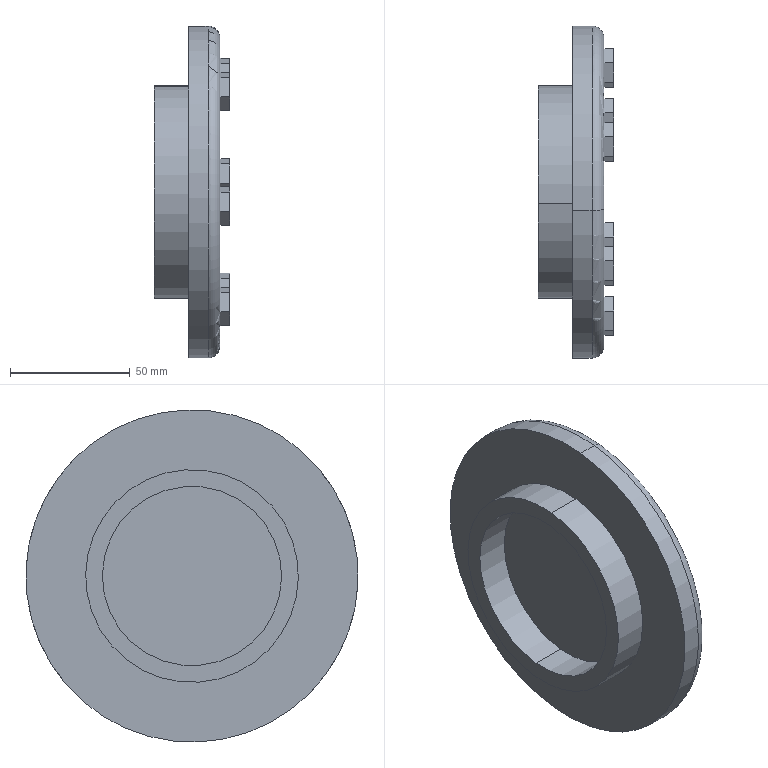Component | SolidWorks | UpperEndCap-1 | 1 solid | 54 faces | volume 225267 mm3 | plane 46 | cylinder 6 | torus 2 | commonest cylinder face diameters 75 x2 139 x2 89 x2